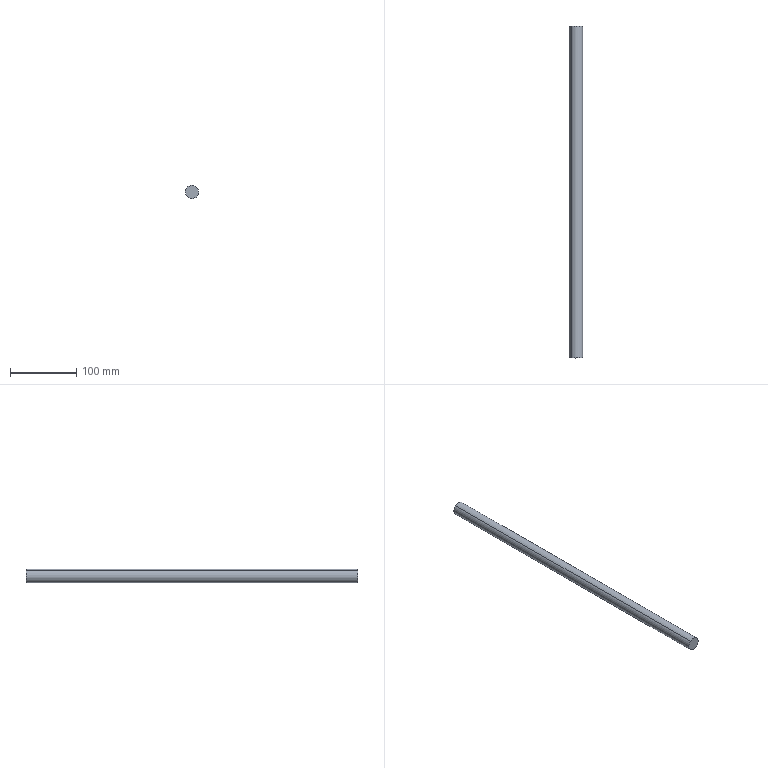Component | SolidWorks | 20OpticalAxis1-1-1 | 1 solid | 8 faces | box 20 x 500 x 20 mm | volume 156338 mm3 | cylinder 4 | cone 2 | plane 2 | commonest cylinder face diameters 6.8 x2 20 x2
build123d program:
from build123d import *

# Parameters (mm, degrees)
SKETCH1_R             = 10
BOSS_EXTRUDE1_DEPTH   = 500
M8_TAPPED_HOLE1_D     = 6.8
M8_TAPPED_HOLE1_DEPTH = 19.75
M8_TAPPED_HOLE1_TIP   = 2.043


with BuildPart() as part:
    # Sketch1 → Boss-Extrude1 (new body)
    with BuildSketch(Plane.XY):
        Circle(SKETCH1_R)
    extrude(amount=BOSS_EXTRUDE1_DEPTH)

    # M8 Tapped Hole1
    with Locations(Plane(origin=(0, 0, 0), x_dir=(-1, 0, 0), z_dir=(0, 0, -1))):
        with Locations((0, 0)):
            Hole(M8_TAPPED_HOLE1_D / 2, depth=M8_TAPPED_HOLE1_DEPTH)
            with Locations((0, 0, -(M8_TAPPED_HOLE1_DEPTH + M8_TAPPED_HOLE1_TIP / 2))):  # 118° drill point
                Cone(0, M8_TAPPED_HOLE1_D / 2, M8_TAPPED_HOLE1_TIP, mode=Mode.SUBTRACT)


solid = part.part

# Placed as in the assembly
solid = solid.moved(Location((-30.965, 500, 663.073), (90, 0, 0)))
STEP:
#1=COLOUR_RGB('',0.7922,0.8196,0.9333);
#2=FILL_AREA_STYLE_COLOUR('',#1);
#3=FILL_AREA_STYLE('',(#2));
#4=SURFACE_STYLE_FILL_AREA(#3);
#5=SURFACE_SIDE_STYLE('',(#4));
#6=SURFACE_STYLE_USAGE(.BOTH.,#5);
#7=PRESENTATION_STYLE_ASSIGNMENT((#6));
#8=CARTESIAN_POINT('',(-1.304,18.907,26.209));
#9=VERTEX_POINT('',#8);
#10=CARTESIAN_POINT('',(-1.134,18.907,26.002));
#11=VERTEX_POINT('',#10);
#12=CARTESIAN_POINT('',(-1.219,18.907,26.105));
#13=DIRECTION('',(-0.,1.,-0.));
#14=DIRECTION('',(0.6334,0.,-0.7739));
#15=AXIS2_PLACEMENT_3D('',#12,#13,#14);
#16=CIRCLE('',#15,0.1339);
#17=EDGE_CURVE('',#9,#11,#16,.T.);
#18=ORIENTED_EDGE('',*,*,#17,.F.);
#19=CARTESIAN_POINT('',(-1.304,19.685,26.209));
#20=VERTEX_POINT('',#19);
#21=CARTESIAN_POINT('',(-1.304,19.685,26.209));
#22=DIRECTION('',(-0.,1.,-0.));
#23=VECTOR('',#22,39.37);
#24=LINE('',#21,#23);
#25=EDGE_CURVE('',#9,#20,#24,.T.);
#26=ORIENTED_EDGE('',*,*,#25,.T.);
#27=CARTESIAN_POINT('',(-1.134,19.685,26.002));
#28=VERTEX_POINT('',#27);
#29=CARTESIAN_POINT('',(-1.219,19.685,26.105));
#30=DIRECTION('',(-0.,1.,-0.));
#31=DIRECTION('',(0.6334,0.,-0.7739));
#32=AXIS2_PLACEMENT_3D('',#29,#30,#31);
#33=CIRCLE('',#32,0.1339);
#34=EDGE_CURVE('',#20,#28,#33,.T.);
#35=ORIENTED_EDGE('',*,*,#34,.T.);
#36=CARTESIAN_POINT('',(-1.134,19.685,26.002));
#37=DIRECTION('',(-0.,1.,-0.));
#38=VECTOR('',#37,39.37);
#39=LINE('',#36,#38);
#40=EDGE_CURVE('',#11,#28,#39,.T.);
#41=ORIENTED_EDGE('',*,*,#40,.F.);
#42=EDGE_LOOP('',(#18,#26,#35,#41));
#43=FACE_OUTER_BOUND('',#42,.T.);
#44=CARTESIAN_POINT('',(-1.219,19.685,26.105));
#45=DIRECTION('',(-0.,1.,-0.));
#46=DIRECTION('',(0.6334,0.,-0.7739));
#47=AXIS2_PLACEMENT_3D('',#44,#45,#46);
#48=CYLINDRICAL_SURFACE('',#47,0.1339);
#49=ADVANCED_FACE('',(#43),#48,.F.);
#50=CARTESIAN_POINT('',(-1.219,18.827,26.105));
#51=VERTEX_POINT('',#50);
#52=CARTESIAN_POINT('',(-1.134,18.907,26.002));
#53=DIRECTION('',(0.5429,0.515,-0.6633));
#54=VECTOR('',#53,39.37);
#55=LINE('',#52,#54);
#56=EDGE_CURVE('',#51,#11,#55,.T.);
#57=ORIENTED_EDGE('',*,*,#56,.F.);
#58=CARTESIAN_POINT('',(-1.304,18.907,26.209));
#59=DIRECTION('',(-0.5429,0.515,0.6633));
#60=VECTOR('',#59,39.37);
#61=LINE('',#58,#60);
#62=EDGE_CURVE('',#51,#9,#61,.T.);
#63=ORIENTED_EDGE('',*,*,#62,.T.);
#64=ORIENTED_EDGE('',*,*,#17,.T.);
#65=EDGE_LOOP('',(#57,#63,#64));
#66=FACE_OUTER_BOUND('',#65,.T.);
#67=CARTESIAN_POINT('',(-1.219,18.907,26.105));
#68=DIRECTION('',(-0.,1.,-0.));
#69=DIRECTION('',(0.6334,0.,-0.7739));
#70=AXIS2_PLACEMENT_3D('',#67,#68,#69);
#71=CONICAL_SURFACE('',#70,0.1339,1.03);
#72=ADVANCED_FACE('',(#66),#71,.F.);
#73=CARTESIAN_POINT('',(-1.468,0.,26.41));
#74=VERTEX_POINT('',#73);
#75=CARTESIAN_POINT('',(-0.9697,0.,25.801));
#76=VERTEX_POINT('',#75);
#77=CARTESIAN_POINT('',(-1.219,0.,26.105));
#78=DIRECTION('',(0.,-1.,0.));
#79=DIRECTION('',(-0.6334,-0.,0.7739));
#80=AXIS2_PLACEMENT_3D('',#77,#78,#79);
#81=CIRCLE('',#80,0.3937);
#82=EDGE_CURVE('',#74,#76,#81,.T.);
#83=ORIENTED_EDGE('',*,*,#82,.F.);
#84=CARTESIAN_POINT('',(-1.468,19.685,26.41));
#85=VERTEX_POINT('',#84);
#86=CARTESIAN_POINT('',(-1.468,0.,26.41));
#87=DIRECTION('',(-0.,1.,-0.));
#88=VECTOR('',#87,39.37);
#89=LINE('',#86,#88);
#90=EDGE_CURVE('',#74,#85,#89,.T.);
#91=ORIENTED_EDGE('',*,*,#90,.T.);
#92=CARTESIAN_POINT('',(-0.9697,19.685,25.801));
#93=VERTEX_POINT('',#92);
#94=CARTESIAN_POINT('',(-1.219,19.685,26.105));
#95=DIRECTION('',(0.,-1.,0.));
#96=DIRECTION('',(-0.6334,0.,0.7739));
#97=AXIS2_PLACEMENT_3D('',#94,#95,#96);
#98=CIRCLE('',#97,0.3937);
#99=EDGE_CURVE('',#85,#93,#98,.T.);
#100=ORIENTED_EDGE('',*,*,#99,.T.);
#101=CARTESIAN_POINT('',(-0.9697,0.,25.801));
#102=DIRECTION('',(-0.,1.,-0.));
#103=VECTOR('',#102,39.37);
#104=LINE('',#101,#103);
#105=EDGE_CURVE('',#76,#93,#104,.T.);
#106=ORIENTED_EDGE('',*,*,#105,.F.);
#107=EDGE_LOOP('',(#83,#91,#100,#106));
#108=FACE_OUTER_BOUND('',#107,.T.);
#109=CARTESIAN_POINT('',(-1.219,0.,26.105));
#110=DIRECTION('',(-0.,1.,-0.));
#111=DIRECTION('',(0.6334,0.,-0.7739));
#112=AXIS2_PLACEMENT_3D('',#109,#110,#111);
#113=CYLINDRICAL_SURFACE('',#112,0.3937);
#114=ADVANCED_FACE('',(#108),#113,.T.);
#115=ORIENTED_EDGE('',*,*,#90,.F.);
#116=CARTESIAN_POINT('',(-1.219,0.,26.105));
#117=DIRECTION('',(0.,-1.,0.));
#118=DIRECTION('',(-0.6334,-0.,0.7739));
#119=AXIS2_PLACEMENT_3D('',#116,#117,#118);
#120=CIRCLE('',#119,0.3937);
#121=EDGE_CURVE('',#76,#74,#120,.T.);
#122=ORIENTED_EDGE('',*,*,#121,.F.);
#123=ORIENTED_EDGE('',*,*,#105,.T.);
#124=CARTESIAN_POINT('',(-1.219,19.685,26.105));
#125=DIRECTION('',(0.,-1.,0.));
#126=DIRECTION('',(-0.6334,0.,0.7739));
#127=AXIS2_PLACEMENT_3D('',#124,#125,#126);
#128=CIRCLE('',#127,0.3937);
#129=EDGE_CURVE('',#93,#85,#128,.T.);
#130=ORIENTED_EDGE('',*,*,#129,.T.);
#131=EDGE_LOOP('',(#115,#122,#123,#130));
#132=FACE_OUTER_BOUND('',#131,.T.);
#133=CARTESIAN_POINT('',(-1.219,0.,26.105));
#134=DIRECTION('',(-0.,1.,-0.));
#135=DIRECTION('',(0.6334,0.,-0.7739));
#136=AXIS2_PLACEMENT_3D('',#133,#134,#135);
#137=CYLINDRICAL_SURFACE('',#136,0.3937);
#138=ADVANCED_FACE('',(#132),#137,.T.);
#139=ORIENTED_EDGE('',*,*,#121,.T.);
#140=ORIENTED_EDGE('',*,*,#82,.T.);
#141=EDGE_LOOP('',(#139,#140));
#142=FACE_OUTER_BOUND('',#141,.T.);
#143=CARTESIAN_POINT('',(-1.219,0.,26.105));
#144=DIRECTION('',(0.,-1.,0.));
#145=DIRECTION('',(-0.6334,-0.,0.7739));
#146=AXIS2_PLACEMENT_3D('',#143,#144,#145);
#147=PLANE('',#146);
#148=ADVANCED_FACE('',(#142),#147,.T.);
#149=CARTESIAN_POINT('',(-1.219,19.685,26.105));
#150=DIRECTION('',(-0.,1.,-0.));
#151=DIRECTION('',(0.6334,0.,-0.7739));
#152=AXIS2_PLACEMENT_3D('',#149,#150,#151);
#153=CIRCLE('',#152,0.1339);
#154=EDGE_CURVE('',#28,#20,#153,.T.);
#155=ORIENTED_EDGE('',*,*,#154,.F.);
#156=ORIENTED_EDGE('',*,*,#34,.F.);
#157=EDGE_LOOP('',(#155,#156));
#158=FACE_BOUND('',#157,.T.);
#159=ORIENTED_EDGE('',*,*,#129,.F.);
#160=ORIENTED_EDGE('',*,*,#99,.F.);
#161=EDGE_LOOP('',(#159,#160));
#162=FACE_OUTER_BOUND('',#161,.T.);
#163=CARTESIAN_POINT('',(-1.219,19.685,26.105));
#164=DIRECTION('',(0.,-1.,0.));
#165=DIRECTION('',(-0.6334,-0.,0.7739));
#166=AXIS2_PLACEMENT_3D('',#163,#164,#165);
#167=PLANE('',#166);
#168=ADVANCED_FACE('',(#158,#162),#167,.F.);
#169=ORIENTED_EDGE('',*,*,#62,.F.);
#170=ORIENTED_EDGE('',*,*,#56,.T.);
#171=CARTESIAN_POINT('',(-1.219,18.907,26.105));
#172=DIRECTION('',(-0.,1.,-0.));
#173=DIRECTION('',(0.6334,0.,-0.7739));
#174=AXIS2_PLACEMENT_3D('',#171,#172,#173);
#175=CIRCLE('',#174,0.1339);
#176=EDGE_CURVE('',#11,#9,#175,.T.);
#177=ORIENTED_EDGE('',*,*,#176,.T.);
#178=EDGE_LOOP('',(#169,#170,#177));
#179=FACE_OUTER_BOUND('',#178,.T.);
#180=CARTESIAN_POINT('',(-1.219,18.907,26.105));
#181=DIRECTION('',(-0.,1.,-0.));
#182=DIRECTION('',(0.6334,0.,-0.7739));
#183=AXIS2_PLACEMENT_3D('',#180,#181,#182);
#184=CONICAL_SURFACE('',#183,0.1339,1.03);
#185=ADVANCED_FACE('',(#179),#184,.F.);
#186=ORIENTED_EDGE('',*,*,#25,.F.);
#187=ORIENTED_EDGE('',*,*,#176,.F.);
#188=ORIENTED_EDGE('',*,*,#40,.T.);
#189=ORIENTED_EDGE('',*,*,#154,.T.);
#190=EDGE_LOOP('',(#186,#187,#188,#189));
#191=FACE_OUTER_BOUND('',#190,.T.);
#192=CARTESIAN_POINT('',(-1.219,19.685,26.105));
#193=DIRECTION('',(-0.,1.,-0.));
#194=DIRECTION('',(0.6334,0.,-0.7739));
#195=AXIS2_PLACEMENT_3D('',#192,#193,#194);
#196=CYLINDRICAL_SURFACE('',#195,0.1339);
#197=ADVANCED_FACE('',(#191),#196,.F.);
#198=CLOSED_SHELL('',(#49,#72,#114,#138,#148,#168,#185,#197));
#199=MANIFOLD_SOLID_BREP('',#198);
#200=STYLED_ITEM('',(#7),#199);
#201=(LENGTH_UNIT()NAMED_UNIT(*)SI_UNIT($,.METRE.));
#202=LENGTH_MEASURE_WITH_UNIT(LENGTH_MEASURE(0.0254),#201);
#203=DIMENSIONAL_EXPONENTS(1.,0.,0.,0.,0.,0.,0.);
#204=(CONVERSION_BASED_UNIT('',#202)LENGTH_UNIT()NAMED_UNIT(#203));
#205=UNCERTAINTY_MEASURE_WITH_UNIT(LENGTH_MEASURE(0.00001),#204,'','');
#206=(NAMED_UNIT(*)PLANE_ANGLE_UNIT()SI_UNIT($,.RADIAN.));
#207=(NAMED_UNIT(*)SI_UNIT($,.STERADIAN.)SOLID_ANGLE_UNIT());
#208=(GEOMETRIC_REPRESENTATION_CONTEXT(3)GLOBAL_UNCERTAINTY_ASSIGNED_CONTEXT((#205))GLOBAL_UNIT_ASSIGNED_CONTEXT((#204,#206,#207))REPRESENTATION_CONTEXT('',''));
#209=MECHANICAL_DESIGN_GEOMETRIC_PRESENTATION_REPRESENTATION('',(#200),#208);
#210=CARTESIAN_POINT('',(0.,0.,0.));
#211=DIRECTION('',(0.,0.,1.));
#212=DIRECTION('',(1.,0.,0.));
#213=AXIS2_PLACEMENT_3D('',#210,#211,#212);
#214=(LENGTH_UNIT()NAMED_UNIT(*)SI_UNIT($,.METRE.));
#215=LENGTH_MEASURE_WITH_UNIT(LENGTH_MEASURE(0.0254),#214);
#216=DIMENSIONAL_EXPONENTS(1.,0.,0.,0.,0.,0.,0.);
#217=(CONVERSION_BASED_UNIT('',#215)LENGTH_UNIT()NAMED_UNIT(#216));
#218=UNCERTAINTY_MEASURE_WITH_UNIT(LENGTH_MEASURE(0.00001),#217,'','');
#219=(NAMED_UNIT(*)PLANE_ANGLE_UNIT()SI_UNIT($,.RADIAN.));
#220=(NAMED_UNIT(*)SI_UNIT($,.STERADIAN.)SOLID_ANGLE_UNIT());
#221=(GEOMETRIC_REPRESENTATION_CONTEXT(3)GLOBAL_UNCERTAINTY_ASSIGNED_CONTEXT((#218))GLOBAL_UNIT_ASSIGNED_CONTEXT((#217,#219,#220))REPRESENTATION_CONTEXT('',''));
#222=ADVANCED_BREP_SHAPE_REPRESENTATION('',(#199,#213),#221);
#223=PRESENTATION_LAYER_ASSIGNMENT('','',(#200));